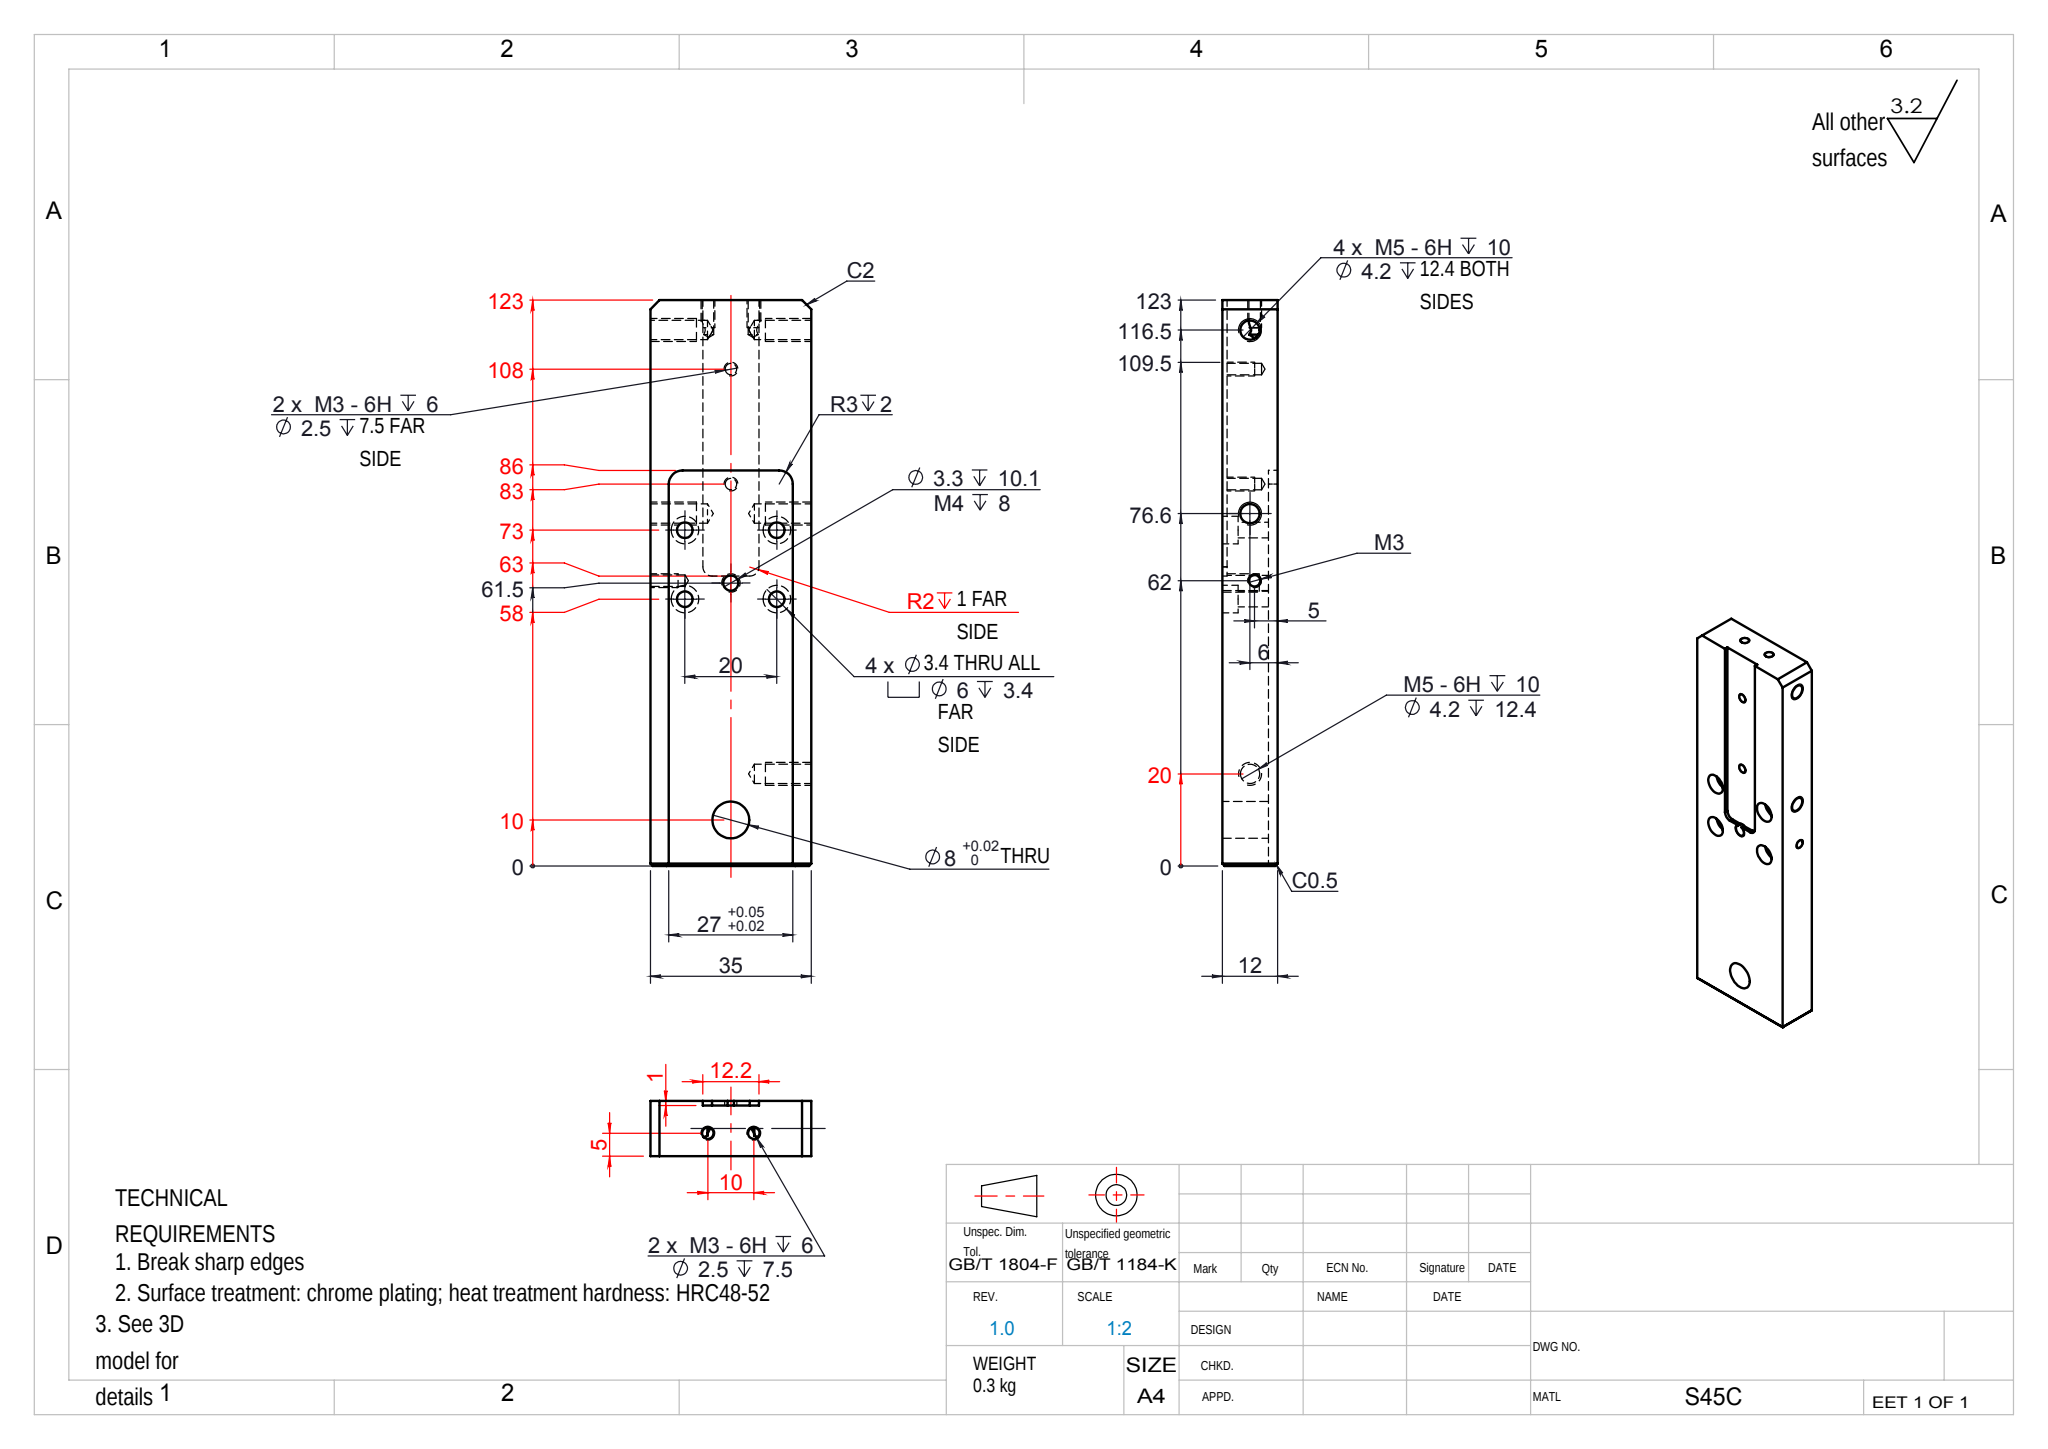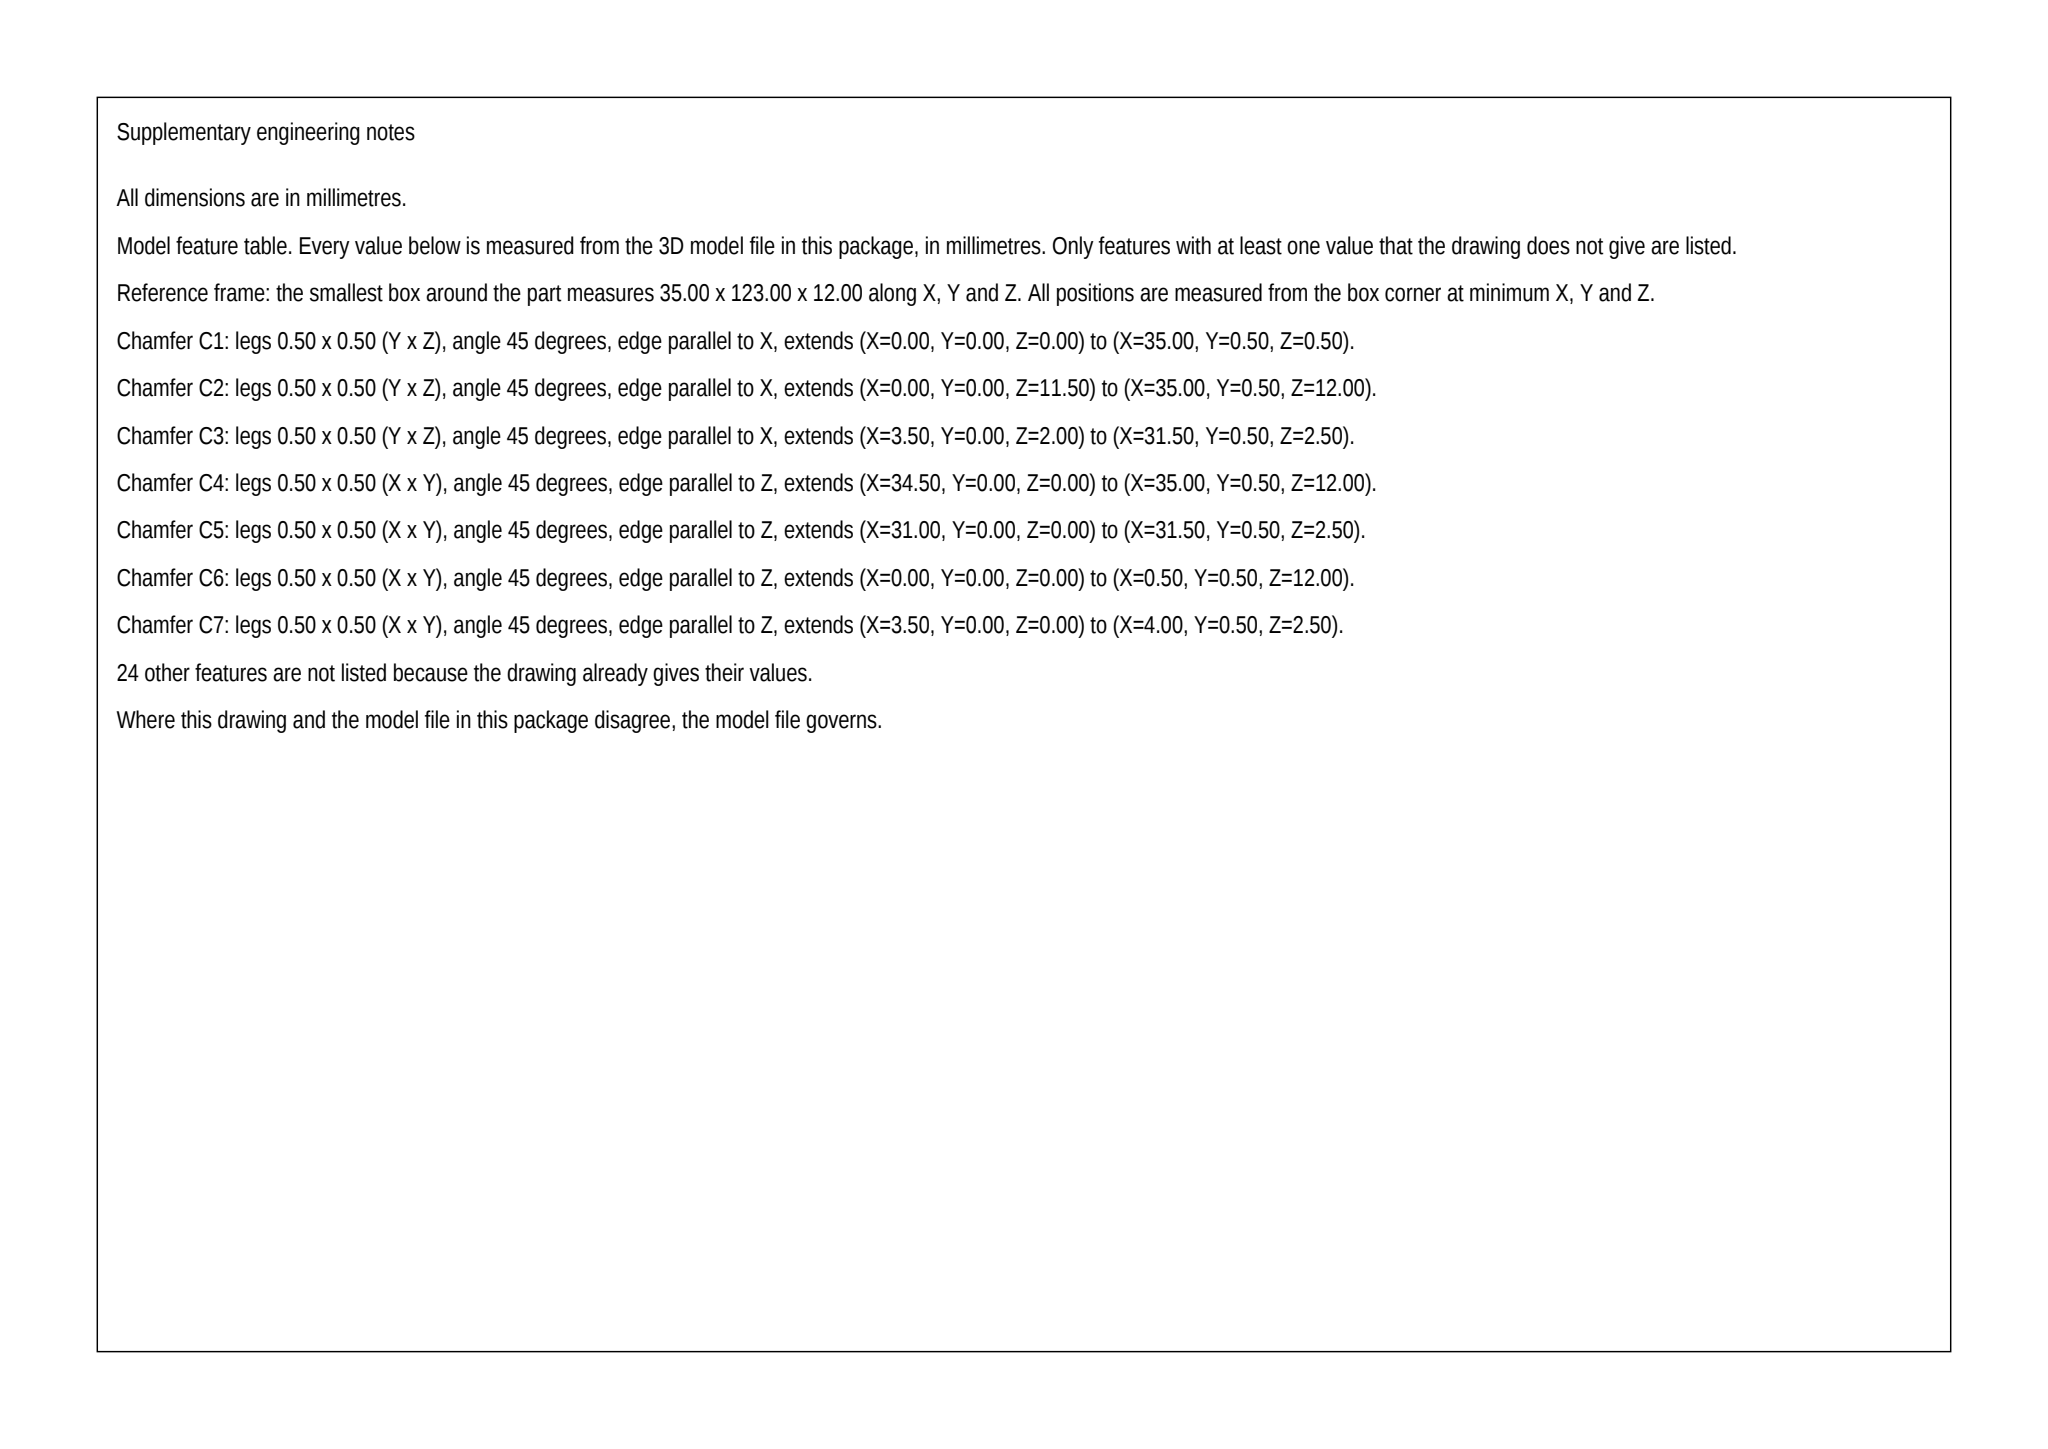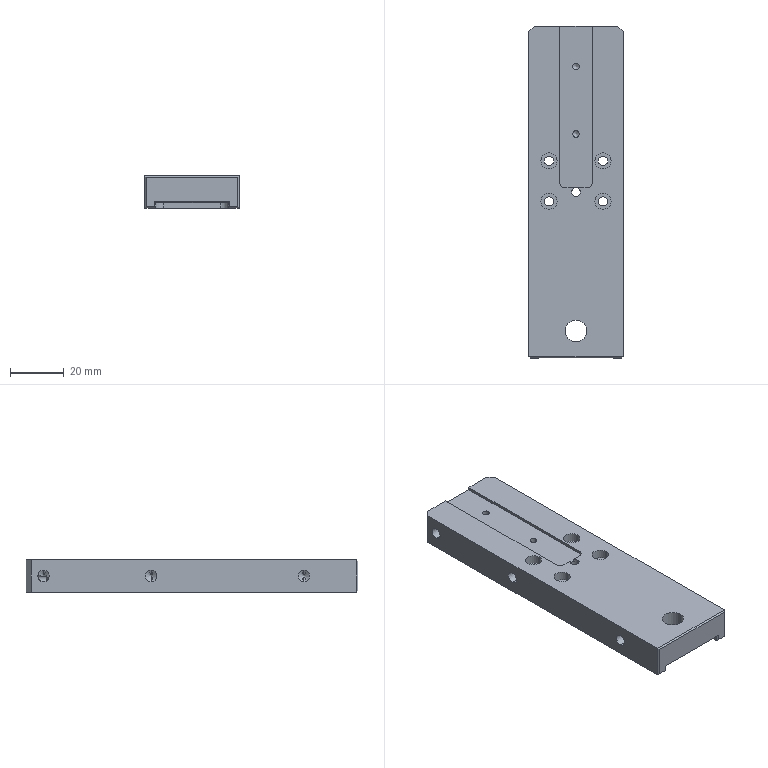Part | SolidWorks | mm | 1 solid | 93 faces | box 35 x 123 x 12 mm | volume 43962 mm3 | cylinder 44 | plane 29 | cone 20 | commonest cylinder face diameters 2.5 x10 4.2 x10 6 x10 3.4 x8 3.3 x2 8 x2 4 x2
Drawing notes:
FRONT RECESS 27 WIDE DP 2, Y0 TO Y86, R3 CORNERS | from the solid: planes x=4.0 & x=31.0 (27 wide), y=86.0; recess floor z=2.0 vs front face z=0; Ø6 len 2 cyls at (7,83) & (28,83) = R3 corners
BACK SLOT 12.2 LG x 4 WIDE, R2, DP 1, CL 65 FROM BOT | from the solid: 2x Ø4 cyl axis z at x13.4 & x21.6, y65, len 1.0; walls x=11.4 & x=23.6 (12.2 apart); floor z=11.0 vs back face z=12.0
2x M3-6H DP 6, Ø2.5 DP 7.5 IN BOT FACE, 10 APART, 5 FROM FRONT | from the solid: 2x Ø2.5 cyl axis y at x12.5 & x22.5 (10 apart), z=5.0, len 7.5, from face y=0; front face z=0
1x M3-6H Ø2.5 DP 7.5 IN SIDE FACE AT Y62, 5 FROM FRONT, 1 SIDE ONLY | from the solid: Ø2.5 cyl axis x at y=62, z=5, len 7.5, single occurrence; 118° drill cone ref 2.5
2x M5-6H DP 10 / Ø4.2 DP 12.4 BOTH SIDES AT Y20, 6 FROM FRONT FACE | from the solid: cyl [4.2,'x',[null,20.0,6.0],12.4] count 2 — tapped from both X faces, axis 6 mm from z=0 front face, Y=20 from bottom edge y=0
M3-6H DP 6, Ø2.5 DP 7.5 IN SIDE FACE AT Y62, Z5 - 1 SIDE ONLY | from the solid: Cylinder Ø2.5, axis X, at Y=62.0, Z=5.0, length 7.5 with 118° drill point cone (ref dia 2.5); thread depth 6 per identical M3-6H ↧6 Ø2.5 ↧7.5 callout on this part
build123d program:
from build123d import *

# Parameters (mm, degrees)
SKETCH1_W                                         = 35
SKETCH1_H                                         = 123
BOSS_EXTRUDE1_DEPTH                               = 6
SKETCH2_W                                         = 27
SKETCH2_H                                         = 86
CUT_EXTRUDE1_DEPTH                                = 2
FILLET1_R                                         = 3
CHAMFER1_SIZE                                     = 2
HOLE_SIZE_ACCORDING_TO_TYPE_1_OF_HEXA_D           = 3.4
HOLE_SIZE_ACCORDING_TO_TYPE_1_OF_HEXA_CBORE_D     = 6
HOLE_SIZE_ACCORDING_TO_TYPE_1_OF_HEXA_CBORE_DEPTH = 3.4
SKETCH7_R                                         = 4
CUT_EXTRUDE4_DEPTH                                = 20
M5_TAPPED_HOLE1_AT_2_COUNT                        = 2
M5_TAPPED_HOLE1_AT_2_PITCH                        = 39.907
M5_TAPPED_HOLE2_D                                 = 4.2
M5_TAPPED_HOLE2_DEPTH                             = 12.4
M5_TAPPED_HOLE2_TIP                               = 1.262
CUT_EXTRUDE5_DEPTH                                = 1
M3_TAPPED_HOLE1_D                                 = 2.5
M3_TAPPED_HOLE1_DEPTH                             = 7.5
M3_TAPPED_HOLE1_TIP                               = 0.7511
CHAMFER3_SIZE                                     = 0.5
M3_TAPPED_HOLE3_D                                 = 2.5
M3_TAPPED_HOLE3_DEPTH                             = 7.5
M3_TAPPED_HOLE3_TIP                               = 0.7511
M3_TAPPED_HOLE4_D                                 = 2.5
M3_TAPPED_HOLE4_DEPTH                             = 7.5
M3_TAPPED_HOLE4_TIP                               = 0.7511
M4_TAPPED_HOLE1_D                                 = 3.3
M4_TAPPED_HOLE1_DEPTH                             = 10.1
M4_TAPPED_HOLE1_TIP                               = 0.9914


with BuildPart() as part:
    # Sketch1 → Boss-Extrude1 (new, symmetric)
    with BuildSketch(Plane.XY):
        Rectangle(SKETCH1_W, SKETCH1_H)
    extrude(amount=BOSS_EXTRUDE1_DEPTH, both=True)

    # Sketch2 → Cut-Extrude1 (cut)
    with BuildSketch(Plane(origin=(0, 0, -6), x_dir=(-1, 0, 0), z_dir=(0, 0, -1))):
        with Locations((0, -18.5)):
            Rectangle(SKETCH2_W, SKETCH2_H)
    extrude(amount=-CUT_EXTRUDE1_DEPTH, mode=Mode.SUBTRACT)

    # Fillet1
    fillet1_edges = [part.edges().sort_by_distance(p)[0] for p in [
        (13.5, 24.5, -5),
        (-13.5, 24.5, -5),
    ]]
    fillet(fillet1_edges, radius=FILLET1_R)

    # Chamfer1
    chamfer1_edges = [part.edges().sort_by_distance(p)[0] for p in [
        (-17.5, 61.5, 0),
        (17.5, 61.5, 0),
    ]]
    chamfer(chamfer1_edges, length=CHAMFER1_SIZE)

    # Hole Size _ according to_ type 1 of Hexa (through all)
    with Locations(Plane.XY.offset(6)):
        with Locations((10, 11.5), (-10, 11.5), (10, -3.5), (-10, -3.5)):
            CounterBoreHole(HOLE_SIZE_ACCORDING_TO_TYPE_1_OF_HEXA_D / 2, HOLE_SIZE_ACCORDING_TO_TYPE_1_OF_HEXA_CBORE_D / 2, HOLE_SIZE_ACCORDING_TO_TYPE_1_OF_HEXA_CBORE_DEPTH)

    # Sketch7 → Cut-Extrude4 (cut)
    with BuildSketch(Plane(origin=(0, 0, -6), x_dir=(-1, 0, 0), z_dir=(0, 0, -1))):
        with Locations((0, -51.5)):
            Circle(SKETCH7_R)
    extrude(amount=-CUT_EXTRUDE4_DEPTH, mode=Mode.SUBTRACT)

    # Sketch9 → M5 Tapped Hole1 (revolve, cut)
    with BuildSketch(Plane(origin=(-17.5, 55, 0), x_dir=(0, 0, 1), z_dir=(0, 1, 0))):
        Polygon((0, 0), (0, 13.662), (2.1, 12.4), (2.1, 0), align=None)
    m5_tapped_hole1 = revolve(axis=Axis((-23.85, 55, 0), (1, 0, 0)), mode=Mode.SUBTRACT)

    # M5 Tapped Hole1 at 2: M5 Tapped Hole1 ×2
    with Locations(*[(0, -i * M5_TAPPED_HOLE1_AT_2_PITCH, 0) for i in range(1, M5_TAPPED_HOLE1_AT_2_COUNT)]):
        add(m5_tapped_hole1, mode=Mode.SUBTRACT)

    # M5 Tapped Hole2
    with Locations(Plane.ZY.offset(17.5)):
        with Locations((0, -41.5)):
            Hole(M5_TAPPED_HOLE2_D / 2, depth=M5_TAPPED_HOLE2_DEPTH)
            with Locations((0, 0, -(M5_TAPPED_HOLE2_DEPTH + M5_TAPPED_HOLE2_TIP / 2))):  # 118° drill point
                Cone(0, M5_TAPPED_HOLE2_D / 2, M5_TAPPED_HOLE2_TIP, mode=Mode.SUBTRACT)

    # Sketch12 → Cut-Extrude5 (cut)
    with BuildSketch(Plane.XY.offset(6)):
        with BuildLine():
            Line((-6.1, 71.5), (6.1, 71.5))
            Line((6.1, 71.5), (6.1, 3.5))
            ThreePointArc((6.1, 3.5), (5.514, 2.086), (4.1, 1.5))
            Line((4.1, 1.5), (-4.1, 1.5))
            ThreePointArc((-4.1, 1.5), (-5.514, 2.086), (-6.1, 3.5))
            Line((-6.1, 3.5), (-6.1, 71.5))
        make_face()
    extrude(amount=-CUT_EXTRUDE5_DEPTH, mode=Mode.SUBTRACT)

    # M3 Tapped Hole1
    with Locations(Plane.XY.offset(5)):
        with Locations((0, 21.5), (0, 46.5)):
            Hole(M3_TAPPED_HOLE1_D / 2, depth=M3_TAPPED_HOLE1_DEPTH)
            with Locations((0, 0, -(M3_TAPPED_HOLE1_DEPTH + M3_TAPPED_HOLE1_TIP / 2))):  # 118° drill point
                Cone(0, M3_TAPPED_HOLE1_D / 2, M3_TAPPED_HOLE1_TIP, mode=Mode.SUBTRACT)

    # Chamfer3
    chamfer3_edges = [part.edges().sort_by_distance(p)[0] for p in [
        (15.5, -61.5, -6),
        (0, -61.5, 6),
        (13.5, -61.5, -5),
        (0, -61.5, -4),
        (-13.5, -61.5, -5),
        (-15.5, -61.5, -6),
        (17.5, -61.5, 0),
        (-17.5, -61.5, 0),
    ]]
    chamfer(chamfer3_edges, length=CHAMFER3_SIZE)

    # Mirror1: M5 Tapped Hole1 across plane
    add(m5_tapped_hole1.mirror(Plane.ZY), mode=Mode.SUBTRACT)

    # Mirror1 copy 1 sketch → Mirror1 copy 1 (revolve, cut)
    with BuildSketch(Plane(origin=(17.5, 15.093, 0), x_dir=(0, 0, 1), z_dir=(0, 1, 0))):
        Polygon((0, 0), (0, -13.662), (2.1, -12.4), (2.1, 0), align=None)
    revolve(axis=Axis((23.85, 15.093, 0), (1, 0, 0)), mode=Mode.SUBTRACT)

    # M3 Tapped Hole3
    with Locations(Plane(origin=(0, 61.5, 0), x_dir=(1, 0, 0), z_dir=(0, 1, 0))):
        with Locations((-5, 1), (5, 1)):
            Hole(M3_TAPPED_HOLE3_D / 2, depth=M3_TAPPED_HOLE3_DEPTH)
            with Locations((0, 0, -(M3_TAPPED_HOLE3_DEPTH + M3_TAPPED_HOLE3_TIP / 2))):  # 118° drill point
                Cone(0, M3_TAPPED_HOLE3_D / 2, M3_TAPPED_HOLE3_TIP, mode=Mode.SUBTRACT)

    # M3 Tapped Hole4
    with Locations(Plane(origin=(17.5, 0, 0), x_dir=(0, 0, -1), z_dir=(1, 0, 0))):
        with Locations((1, 0.5)):
            Hole(M3_TAPPED_HOLE4_D / 2, depth=M3_TAPPED_HOLE4_DEPTH)
            with Locations((0, 0, -(M3_TAPPED_HOLE4_DEPTH + M3_TAPPED_HOLE4_TIP / 2))):  # 118° drill point
                Cone(0, M3_TAPPED_HOLE4_D / 2, M3_TAPPED_HOLE4_TIP, mode=Mode.SUBTRACT)

    # M4 Tapped Hole1
    with Locations(Plane.XY.offset(6)):
        with Locations((0, 0)):
            Hole(M4_TAPPED_HOLE1_D / 2, depth=M4_TAPPED_HOLE1_DEPTH)
            with Locations((0, 0, -(M4_TAPPED_HOLE1_DEPTH + M4_TAPPED_HOLE1_TIP / 2))):  # 118° drill point
                Cone(0, M4_TAPPED_HOLE1_D / 2, M4_TAPPED_HOLE1_TIP, mode=Mode.SUBTRACT)


solid = part.part